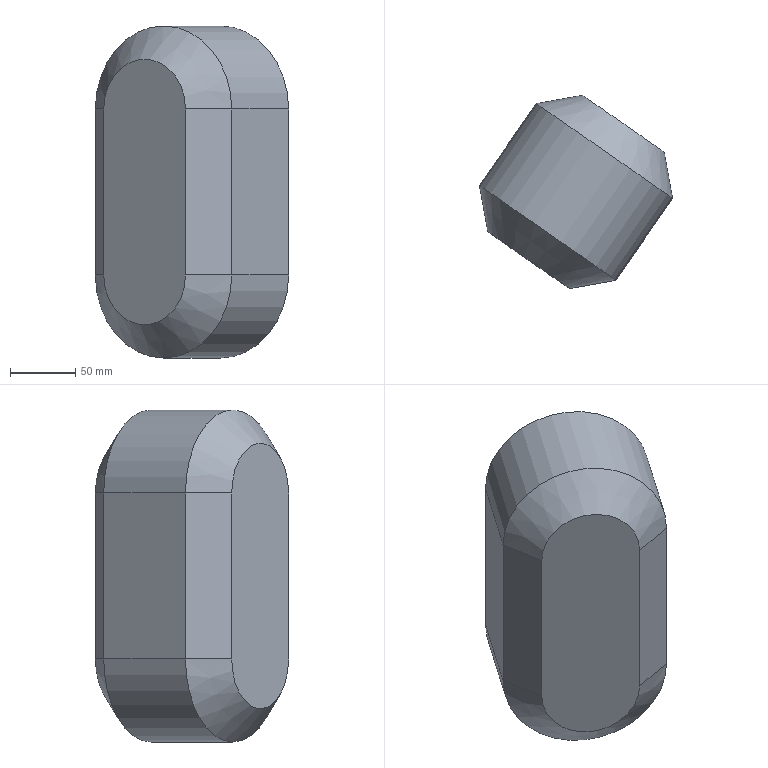Component | NX | 14 | 1 solid | 14 faces | volume 3270222 mm3 | plane 8 | cone 4 | cylinder 2 | commonest cylinder face diameters 127 x2